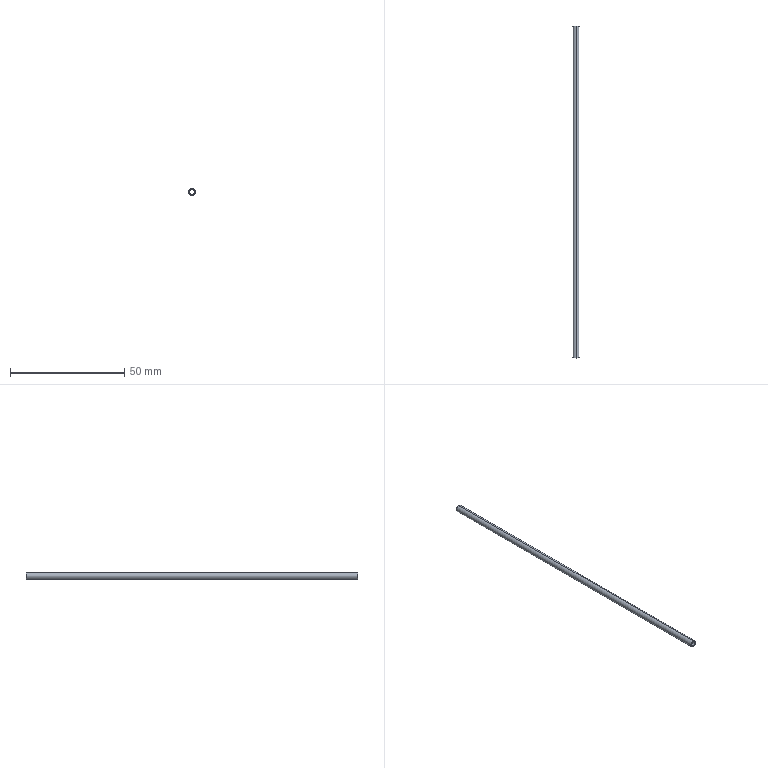Component | SolidWorks | PenRefillTube-1 | 1 solid | 6 faces | box 3 x 145 x 3 mm | volume 569 mm3 | cylinder 4 | plane 2 | commonest cylinder face diameters 2 x2 3 x2
build123d program:
from build123d import *

# Parameters (mm, degrees)
SKETCH1_R           = 1.5
BOSS_EXTRUDE1_DEPTH = 145
SHELL1_T            = -0.5


with BuildPart() as part:
    # Sketch1 → Boss-Extrude1 (new body)
    with BuildSketch(Plane(origin=(0, 0, 0), x_dir=(1, 0, 0), z_dir=(0, 1, 0))):
        with Locations(Location((0, 0, 0), (0, 0, 270))):
            Circle(SKETCH1_R)
    extrude(amount=BOSS_EXTRUDE1_DEPTH)

    # Shell1
    shell1_openings = [part.faces().sort_by_distance(p)[0] for p in [
        (0, 145, 0),
        (0, 0, 0),
    ]]
    offset(amount=SHELL1_T, openings=shell1_openings, kind=Kind.INTERSECTION)


solid = part.part

# Placed as in the assembly
solid = solid.moved(Location((-56.698, -104.764, -29.961), (0, 0, 0)))
STEP:
#1=CARTESIAN_POINT('',(-2.232,1.584,-1.14));
#2=VERTEX_POINT('',#1);
#3=CARTESIAN_POINT('',(-2.232,1.584,-1.219));
#4=VERTEX_POINT('',#3);
#5=CARTESIAN_POINT('',(-2.232,1.584,-1.18));
#6=DIRECTION('',(0.,1.,0.));
#7=DIRECTION('',(0.,0.,-1.));
#8=AXIS2_PLACEMENT_3D('',#5,#6,#7);
#9=CIRCLE('',#8,0.03937);
#10=EDGE_CURVE('',#2,#4,#9,.T.);
#11=ORIENTED_EDGE('',*,*,#10,.T.);
#12=CARTESIAN_POINT('',(-2.232,-4.125,-1.219));
#13=VERTEX_POINT('',#12);
#14=CARTESIAN_POINT('',(-2.232,1.584,-1.219));
#15=DIRECTION('',(0.,-1.,0.));
#16=VECTOR('',#15,39.37);
#17=LINE('',#14,#16);
#18=EDGE_CURVE('',#4,#13,#17,.T.);
#19=ORIENTED_EDGE('',*,*,#18,.T.);
#20=CARTESIAN_POINT('',(-2.232,-4.125,-1.14));
#21=VERTEX_POINT('',#20);
#22=CARTESIAN_POINT('',(-2.232,-4.125,-1.18));
#23=DIRECTION('',(0.,1.,0.));
#24=DIRECTION('',(0.,0.,-1.));
#25=AXIS2_PLACEMENT_3D('',#22,#23,#24);
#26=CIRCLE('',#25,0.03937);
#27=EDGE_CURVE('',#21,#13,#26,.T.);
#28=ORIENTED_EDGE('',*,*,#27,.F.);
#29=CARTESIAN_POINT('',(-2.232,1.584,-1.14));
#30=DIRECTION('',(0.,-1.,0.));
#31=VECTOR('',#30,39.37);
#32=LINE('',#29,#31);
#33=EDGE_CURVE('',#2,#21,#32,.T.);
#34=ORIENTED_EDGE('',*,*,#33,.F.);
#35=EDGE_LOOP('',(#11,#19,#28,#34));
#36=FACE_OUTER_BOUND('',#35,.T.);
#37=CARTESIAN_POINT('',(-2.232,1.584,-1.18));
#38=DIRECTION('',(0.,-1.,0.));
#39=DIRECTION('',(0.,0.,1.));
#40=AXIS2_PLACEMENT_3D('',#37,#38,#39);
#41=CYLINDRICAL_SURFACE('',#40,0.03937);
#42=ADVANCED_FACE('',(#36),#41,.F.);
#43=CARTESIAN_POINT('',(-2.232,1.584,-1.239));
#44=VERTEX_POINT('',#43);
#45=CARTESIAN_POINT('',(-2.232,1.584,-1.121));
#46=VERTEX_POINT('',#45);
#47=CARTESIAN_POINT('',(-2.232,1.584,-1.18));
#48=DIRECTION('',(0.,1.,0.));
#49=DIRECTION('',(0.,0.,-1.));
#50=AXIS2_PLACEMENT_3D('',#47,#48,#49);
#51=CIRCLE('',#50,0.05906);
#52=EDGE_CURVE('',#44,#46,#51,.T.);
#53=ORIENTED_EDGE('',*,*,#52,.F.);
#54=CARTESIAN_POINT('',(-2.232,-4.125,-1.239));
#55=VERTEX_POINT('',#54);
#56=CARTESIAN_POINT('',(-2.232,1.584,-1.239));
#57=DIRECTION('',(0.,-1.,0.));
#58=VECTOR('',#57,39.37);
#59=LINE('',#56,#58);
#60=EDGE_CURVE('',#44,#55,#59,.T.);
#61=ORIENTED_EDGE('',*,*,#60,.T.);
#62=CARTESIAN_POINT('',(-2.232,-4.125,-1.121));
#63=VERTEX_POINT('',#62);
#64=CARTESIAN_POINT('',(-2.232,-4.125,-1.18));
#65=DIRECTION('',(0.,1.,0.));
#66=DIRECTION('',(0.,0.,-1.));
#67=AXIS2_PLACEMENT_3D('',#64,#65,#66);
#68=CIRCLE('',#67,0.05906);
#69=EDGE_CURVE('',#55,#63,#68,.T.);
#70=ORIENTED_EDGE('',*,*,#69,.T.);
#71=CARTESIAN_POINT('',(-2.232,1.584,-1.121));
#72=DIRECTION('',(0.,-1.,0.));
#73=VECTOR('',#72,39.37);
#74=LINE('',#71,#73);
#75=EDGE_CURVE('',#46,#63,#74,.T.);
#76=ORIENTED_EDGE('',*,*,#75,.F.);
#77=EDGE_LOOP('',(#53,#61,#70,#76));
#78=FACE_OUTER_BOUND('',#77,.T.);
#79=CARTESIAN_POINT('',(-2.232,1.584,-1.18));
#80=DIRECTION('',(0.,-1.,0.));
#81=DIRECTION('',(0.,0.,1.));
#82=AXIS2_PLACEMENT_3D('',#79,#80,#81);
#83=CYLINDRICAL_SURFACE('',#82,0.05906);
#84=ADVANCED_FACE('',(#78),#83,.T.);
#85=ORIENTED_EDGE('',*,*,#60,.F.);
#86=CARTESIAN_POINT('',(-2.232,1.584,-1.18));
#87=DIRECTION('',(0.,1.,0.));
#88=DIRECTION('',(0.,0.,-1.));
#89=AXIS2_PLACEMENT_3D('',#86,#87,#88);
#90=CIRCLE('',#89,0.05906);
#91=EDGE_CURVE('',#46,#44,#90,.T.);
#92=ORIENTED_EDGE('',*,*,#91,.F.);
#93=ORIENTED_EDGE('',*,*,#75,.T.);
#94=CARTESIAN_POINT('',(-2.232,-4.125,-1.18));
#95=DIRECTION('',(0.,1.,0.));
#96=DIRECTION('',(0.,0.,-1.));
#97=AXIS2_PLACEMENT_3D('',#94,#95,#96);
#98=CIRCLE('',#97,0.05906);
#99=EDGE_CURVE('',#63,#55,#98,.T.);
#100=ORIENTED_EDGE('',*,*,#99,.T.);
#101=EDGE_LOOP('',(#85,#92,#93,#100));
#102=FACE_OUTER_BOUND('',#101,.T.);
#103=CARTESIAN_POINT('',(-2.232,1.584,-1.18));
#104=DIRECTION('',(0.,-1.,0.));
#105=DIRECTION('',(0.,0.,1.));
#106=AXIS2_PLACEMENT_3D('',#103,#104,#105);
#107=CYLINDRICAL_SURFACE('',#106,0.05906);
#108=ADVANCED_FACE('',(#102),#107,.T.);
#109=ORIENTED_EDGE('',*,*,#10,.F.);
#110=CARTESIAN_POINT('',(-2.232,1.584,-1.18));
#111=DIRECTION('',(0.,1.,0.));
#112=DIRECTION('',(0.,0.,-1.));
#113=AXIS2_PLACEMENT_3D('',#110,#111,#112);
#114=CIRCLE('',#113,0.03937);
#115=EDGE_CURVE('',#4,#2,#114,.T.);
#116=ORIENTED_EDGE('',*,*,#115,.F.);
#117=EDGE_LOOP('',(#109,#116));
#118=FACE_BOUND('',#117,.T.);
#119=ORIENTED_EDGE('',*,*,#91,.T.);
#120=ORIENTED_EDGE('',*,*,#52,.T.);
#121=EDGE_LOOP('',(#119,#120));
#122=FACE_OUTER_BOUND('',#121,.T.);
#123=CARTESIAN_POINT('',(-2.232,1.584,-1.18));
#124=DIRECTION('',(0.,1.,0.));
#125=DIRECTION('',(0.,0.,-1.));
#126=AXIS2_PLACEMENT_3D('',#123,#124,#125);
#127=PLANE('',#126);
#128=ADVANCED_FACE('',(#118,#122),#127,.T.);
#129=ORIENTED_EDGE('',*,*,#27,.T.);
#130=CARTESIAN_POINT('',(-2.232,-4.125,-1.18));
#131=DIRECTION('',(0.,1.,0.));
#132=DIRECTION('',(0.,0.,-1.));
#133=AXIS2_PLACEMENT_3D('',#130,#131,#132);
#134=CIRCLE('',#133,0.03937);
#135=EDGE_CURVE('',#13,#21,#134,.T.);
#136=ORIENTED_EDGE('',*,*,#135,.T.);
#137=EDGE_LOOP('',(#129,#136));
#138=FACE_BOUND('',#137,.T.);
#139=ORIENTED_EDGE('',*,*,#99,.F.);
#140=ORIENTED_EDGE('',*,*,#69,.F.);
#141=EDGE_LOOP('',(#139,#140));
#142=FACE_OUTER_BOUND('',#141,.T.);
#143=CARTESIAN_POINT('',(-2.232,-4.125,-1.18));
#144=DIRECTION('',(0.,1.,0.));
#145=DIRECTION('',(0.,0.,-1.));
#146=AXIS2_PLACEMENT_3D('',#143,#144,#145);
#147=PLANE('',#146);
#148=ADVANCED_FACE('',(#138,#142),#147,.F.);
#149=ORIENTED_EDGE('',*,*,#18,.F.);
#150=ORIENTED_EDGE('',*,*,#115,.T.);
#151=ORIENTED_EDGE('',*,*,#33,.T.);
#152=ORIENTED_EDGE('',*,*,#135,.F.);
#153=EDGE_LOOP('',(#149,#150,#151,#152));
#154=FACE_OUTER_BOUND('',#153,.T.);
#155=CARTESIAN_POINT('',(-2.232,1.584,-1.18));
#156=DIRECTION('',(0.,-1.,0.));
#157=DIRECTION('',(0.,0.,1.));
#158=AXIS2_PLACEMENT_3D('',#155,#156,#157);
#159=CYLINDRICAL_SURFACE('',#158,0.03937);
#160=ADVANCED_FACE('',(#154),#159,.F.);
#161=CLOSED_SHELL('',(#42,#84,#108,#128,#148,#160));
#162=MANIFOLD_SOLID_BREP('',#161);
#163=CARTESIAN_POINT('',(0.,0.,0.));
#164=DIRECTION('',(0.,0.,1.));
#165=DIRECTION('',(1.,0.,0.));
#166=AXIS2_PLACEMENT_3D('',#163,#164,#165);
#167=(LENGTH_UNIT()NAMED_UNIT(*)SI_UNIT($,.METRE.));
#168=LENGTH_MEASURE_WITH_UNIT(LENGTH_MEASURE(0.0254),#167);
#169=DIMENSIONAL_EXPONENTS(1.,0.,0.,0.,0.,0.,0.);
#170=(CONVERSION_BASED_UNIT('',#168)LENGTH_UNIT()NAMED_UNIT(#169));
#171=UNCERTAINTY_MEASURE_WITH_UNIT(LENGTH_MEASURE(0.00001),#170,'','');
#172=(NAMED_UNIT(*)PLANE_ANGLE_UNIT()SI_UNIT($,.RADIAN.));
#173=(NAMED_UNIT(*)SI_UNIT($,.STERADIAN.)SOLID_ANGLE_UNIT());
#174=(GEOMETRIC_REPRESENTATION_CONTEXT(3)GLOBAL_UNCERTAINTY_ASSIGNED_CONTEXT((#171))GLOBAL_UNIT_ASSIGNED_CONTEXT((#170,#172,#173))REPRESENTATION_CONTEXT('',''));
#175=ADVANCED_BREP_SHAPE_REPRESENTATION('',(#162,#166),#174);
#176=COLOUR_RGB('',0.7922,0.8196,0.9333);
#177=FILL_AREA_STYLE_COLOUR('',#176);
#178=FILL_AREA_STYLE('',(#177));
#179=SURFACE_STYLE_FILL_AREA(#178);
#180=SURFACE_SIDE_STYLE('',(#179));
#181=SURFACE_STYLE_USAGE(.BOTH.,#180);
#182=PRESENTATION_STYLE_ASSIGNMENT((#181));
#183=STYLED_ITEM('',(#182),#162);
#184=PRESENTATION_LAYER_ASSIGNMENT('','',(#183));
#185=(LENGTH_UNIT()NAMED_UNIT(*)SI_UNIT($,.METRE.));
#186=LENGTH_MEASURE_WITH_UNIT(LENGTH_MEASURE(0.0254),#185);
#187=DIMENSIONAL_EXPONENTS(1.,0.,0.,0.,0.,0.,0.);
#188=(CONVERSION_BASED_UNIT('',#186)LENGTH_UNIT()NAMED_UNIT(#187));
#189=UNCERTAINTY_MEASURE_WITH_UNIT(LENGTH_MEASURE(0.00001),#188,'','');
#190=(NAMED_UNIT(*)PLANE_ANGLE_UNIT()SI_UNIT($,.RADIAN.));
#191=(NAMED_UNIT(*)SI_UNIT($,.STERADIAN.)SOLID_ANGLE_UNIT());
#192=(GEOMETRIC_REPRESENTATION_CONTEXT(3)GLOBAL_UNCERTAINTY_ASSIGNED_CONTEXT((#189))GLOBAL_UNIT_ASSIGNED_CONTEXT((#188,#190,#191))REPRESENTATION_CONTEXT('',''));
#193=MECHANICAL_DESIGN_GEOMETRIC_PRESENTATION_REPRESENTATION('',(#183),#192);